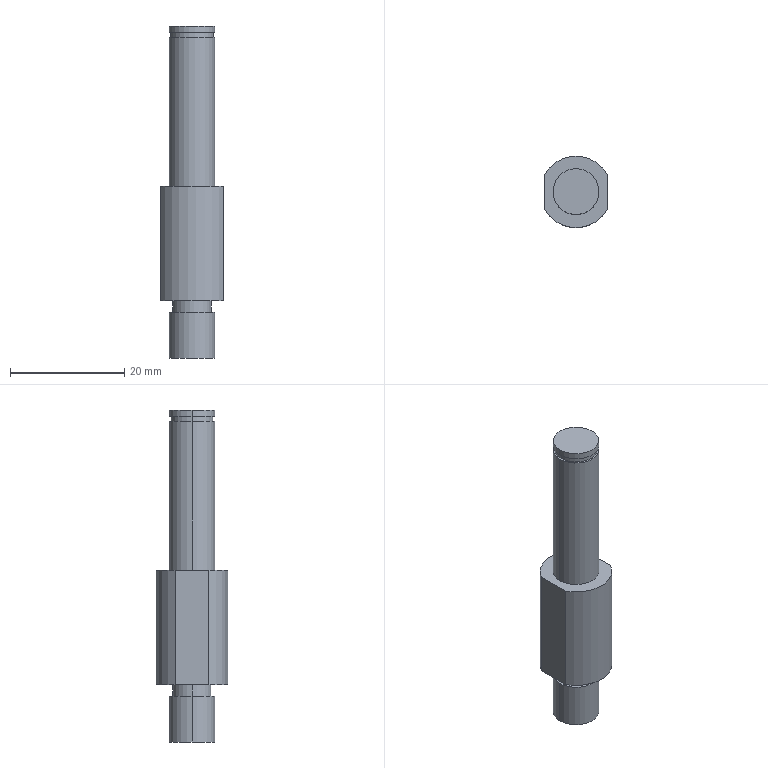Component | SolidWorks | JL001-03-03-1_JL001-03-03-001-1 | 1 solid | 21 faces | box 11 x 12.5 x 58 mm | volume 4210 mm3 | cylinder 12 | plane 9 | commonest cylinder face diameters 8 x6 6.8 x2 7.4 x2 12.5 x2
build123d program:
from build123d import *

# Parameters (mm, degrees)
SKETCH6_OUTSIDE_W   = 26.626
SKETCH6_OUTSIDE_H   = 26.626
SKETCH6_OUTSIDE_W_2 = 19.7
SKETCH6_OUTSIDE_H_2 = 11
CUT_EXTRUDE2_DEPTH  = 32.275


with BuildPart() as part:
    # Sketch1 → Revolve1 (revolve)
    with BuildSketch(Plane.XY, mode=Mode.PRIVATE) as revolve1_sk:
        Polygon((0, 58), (4, 58), (4, 56.9), (3.7, 56.9), (3.7, 56), (4, 56), (4, 30), (6.25, 30), (6.25, 10), (3.4, 10), (3.4, 8), (4, 8), (4, 0), (0, 0), align=None)
    revolve(revolve1_sk.sketch.rotate(Axis((0, 0, 0), (0, 1, 0)), 90), axis=Axis((0, 0, 0), (0, 1, 0)))

    # Sketch6 outside → Cut-Extrude2 (cut, through all)
    with BuildSketch(Plane(origin=(0, 30, 0), x_dir=(1, 0, 0), z_dir=(0, 1, 0))):
        Rectangle(SKETCH6_OUTSIDE_W, SKETCH6_OUTSIDE_H)
        Rectangle(SKETCH6_OUTSIDE_W_2, SKETCH6_OUTSIDE_H_2, mode=Mode.SUBTRACT)
    extrude(amount=-CUT_EXTRUDE2_DEPTH, mode=Mode.SUBTRACT)


solid = part.part

# Placed as in the assembly
solid = solid.moved(Location((15, 27.5, -2.5), (90, -90, 0)))
STEP:
#1=COLOUR_RGB('',0.7922,0.8196,0.9333);
#2=FILL_AREA_STYLE_COLOUR('',#1);
#3=FILL_AREA_STYLE('',(#2));
#4=SURFACE_STYLE_FILL_AREA(#3);
#5=SURFACE_SIDE_STYLE('',(#4));
#6=SURFACE_STYLE_USAGE(.BOTH.,#5);
#7=PRESENTATION_STYLE_ASSIGNMENT((#6));
#8=CARTESIAN_POINT('',(0.748,1.083,0.2165));
#9=VERTEX_POINT('',#8);
#10=CARTESIAN_POINT('',(0.4331,1.083,0.2165));
#11=VERTEX_POINT('',#10);
#12=CARTESIAN_POINT('',(0.5906,1.083,0.2165));
#13=DIRECTION('',(0.,0.,-1.));
#14=DIRECTION('',(1.,0.,0.));
#15=AXIS2_PLACEMENT_3D('',#12,#13,#14);
#16=CIRCLE('',#15,0.1575);
#17=EDGE_CURVE('',#9,#11,#16,.T.);
#18=ORIENTED_EDGE('',*,*,#17,.T.);
#19=CARTESIAN_POINT('',(0.4331,1.083,-0.09843));
#20=VERTEX_POINT('',#19);
#21=CARTESIAN_POINT('',(0.4331,1.083,-0.09843));
#22=DIRECTION('',(0.,0.,-1.));
#23=VECTOR('',#22,39.37);
#24=LINE('',#21,#23);
#25=EDGE_CURVE('',#11,#20,#24,.T.);
#26=ORIENTED_EDGE('',*,*,#25,.T.);
#27=CARTESIAN_POINT('',(0.748,1.083,-0.09843));
#28=VERTEX_POINT('',#27);
#29=CARTESIAN_POINT('',(0.5906,1.083,-0.09843));
#30=DIRECTION('',(0.,0.,-1.));
#31=DIRECTION('',(1.,0.,0.));
#32=AXIS2_PLACEMENT_3D('',#29,#30,#31);
#33=CIRCLE('',#32,0.1575);
#34=EDGE_CURVE('',#28,#20,#33,.T.);
#35=ORIENTED_EDGE('',*,*,#34,.F.);
#36=CARTESIAN_POINT('',(0.748,1.083,-0.09843));
#37=DIRECTION('',(0.,0.,-1.));
#38=VECTOR('',#37,39.37);
#39=LINE('',#36,#38);
#40=EDGE_CURVE('',#9,#28,#39,.T.);
#41=ORIENTED_EDGE('',*,*,#40,.F.);
#42=EDGE_LOOP('',(#18,#26,#35,#41));
#43=FACE_OUTER_BOUND('',#42,.T.);
#44=CARTESIAN_POINT('',(0.5906,1.083,-0.09843));
#45=DIRECTION('',(0.,0.,-1.));
#46=DIRECTION('',(1.,0.,0.));
#47=AXIS2_PLACEMENT_3D('',#44,#45,#46);
#48=CYLINDRICAL_SURFACE('',#47,0.1575);
#49=ADVANCED_FACE('',(#43),#48,.T.);
#50=CARTESIAN_POINT('',(0.7244,1.083,0.2953));
#51=VERTEX_POINT('',#50);
#52=CARTESIAN_POINT('',(0.4567,1.083,0.2953));
#53=VERTEX_POINT('',#52);
#54=CARTESIAN_POINT('',(0.5906,1.083,0.2953));
#55=DIRECTION('',(0.,0.,-1.));
#56=DIRECTION('',(1.,0.,0.));
#57=AXIS2_PLACEMENT_3D('',#54,#55,#56);
#58=CIRCLE('',#57,0.1339);
#59=EDGE_CURVE('',#51,#53,#58,.T.);
#60=ORIENTED_EDGE('',*,*,#59,.T.);
#61=CARTESIAN_POINT('',(0.4567,1.083,0.2165));
#62=VERTEX_POINT('',#61);
#63=CARTESIAN_POINT('',(0.4567,1.083,-0.09843));
#64=DIRECTION('',(0.,0.,-1.));
#65=VECTOR('',#64,39.37);
#66=LINE('',#63,#65);
#67=EDGE_CURVE('',#53,#62,#66,.T.);
#68=ORIENTED_EDGE('',*,*,#67,.T.);
#69=CARTESIAN_POINT('',(0.7244,1.083,0.2165));
#70=VERTEX_POINT('',#69);
#71=CARTESIAN_POINT('',(0.5906,1.083,0.2165));
#72=DIRECTION('',(0.,0.,-1.));
#73=DIRECTION('',(1.,0.,0.));
#74=AXIS2_PLACEMENT_3D('',#71,#72,#73);
#75=CIRCLE('',#74,0.1339);
#76=EDGE_CURVE('',#70,#62,#75,.T.);
#77=ORIENTED_EDGE('',*,*,#76,.F.);
#78=CARTESIAN_POINT('',(0.7244,1.083,-0.09843));
#79=DIRECTION('',(0.,0.,-1.));
#80=VECTOR('',#79,39.37);
#81=LINE('',#78,#80);
#82=EDGE_CURVE('',#51,#70,#81,.T.);
#83=ORIENTED_EDGE('',*,*,#82,.F.);
#84=EDGE_LOOP('',(#60,#68,#77,#83));
#85=FACE_OUTER_BOUND('',#84,.T.);
#86=CARTESIAN_POINT('',(0.5906,1.083,-0.09843));
#87=DIRECTION('',(0.,0.,-1.));
#88=DIRECTION('',(1.,0.,0.));
#89=AXIS2_PLACEMENT_3D('',#86,#87,#88);
#90=CYLINDRICAL_SURFACE('',#89,0.1339);
#91=ADVANCED_FACE('',(#85),#90,.T.);
#92=CARTESIAN_POINT('',(0.748,1.083,2.106));
#93=VERTEX_POINT('',#92);
#94=CARTESIAN_POINT('',(0.4331,1.083,2.106));
#95=VERTEX_POINT('',#94);
#96=CARTESIAN_POINT('',(0.5906,1.083,2.106));
#97=DIRECTION('',(0.,0.,-1.));
#98=DIRECTION('',(1.,0.,0.));
#99=AXIS2_PLACEMENT_3D('',#96,#97,#98);
#100=CIRCLE('',#99,0.1575);
#101=EDGE_CURVE('',#93,#95,#100,.T.);
#102=ORIENTED_EDGE('',*,*,#101,.T.);
#103=CARTESIAN_POINT('',(0.4331,1.083,1.083));
#104=VERTEX_POINT('',#103);
#105=CARTESIAN_POINT('',(0.4331,1.083,-0.09843));
#106=DIRECTION('',(0.,0.,-1.));
#107=VECTOR('',#106,39.37);
#108=LINE('',#105,#107);
#109=EDGE_CURVE('',#95,#104,#108,.T.);
#110=ORIENTED_EDGE('',*,*,#109,.T.);
#111=CARTESIAN_POINT('',(0.748,1.083,1.083));
#112=VERTEX_POINT('',#111);
#113=CARTESIAN_POINT('',(0.5906,1.083,1.083));
#114=DIRECTION('',(0.,0.,-1.));
#115=DIRECTION('',(1.,0.,0.));
#116=AXIS2_PLACEMENT_3D('',#113,#114,#115);
#117=CIRCLE('',#116,0.1575);
#118=EDGE_CURVE('',#112,#104,#117,.T.);
#119=ORIENTED_EDGE('',*,*,#118,.F.);
#120=CARTESIAN_POINT('',(0.748,1.083,-0.09843));
#121=DIRECTION('',(0.,0.,-1.));
#122=VECTOR('',#121,39.37);
#123=LINE('',#120,#122);
#124=EDGE_CURVE('',#93,#112,#123,.T.);
#125=ORIENTED_EDGE('',*,*,#124,.F.);
#126=EDGE_LOOP('',(#102,#110,#119,#125));
#127=FACE_OUTER_BOUND('',#126,.T.);
#128=CARTESIAN_POINT('',(0.5906,1.083,-0.09843));
#129=DIRECTION('',(0.,0.,-1.));
#130=DIRECTION('',(1.,0.,0.));
#131=AXIS2_PLACEMENT_3D('',#128,#129,#130);
#132=CYLINDRICAL_SURFACE('',#131,0.1575);
#133=ADVANCED_FACE('',(#127),#132,.T.);
#134=CARTESIAN_POINT('',(0.7362,1.083,2.142));
#135=VERTEX_POINT('',#134);
#136=CARTESIAN_POINT('',(0.4449,1.083,2.142));
#137=VERTEX_POINT('',#136);
#138=CARTESIAN_POINT('',(0.5906,1.083,2.142));
#139=DIRECTION('',(0.,0.,-1.));
#140=DIRECTION('',(1.,0.,0.));
#141=AXIS2_PLACEMENT_3D('',#138,#139,#140);
#142=CIRCLE('',#141,0.1457);
#143=EDGE_CURVE('',#135,#137,#142,.T.);
#144=ORIENTED_EDGE('',*,*,#143,.T.);
#145=CARTESIAN_POINT('',(0.4449,1.083,2.106));
#146=VERTEX_POINT('',#145);
#147=CARTESIAN_POINT('',(0.4449,1.083,-0.09843));
#148=DIRECTION('',(0.,0.,-1.));
#149=VECTOR('',#148,39.37);
#150=LINE('',#147,#149);
#151=EDGE_CURVE('',#137,#146,#150,.T.);
#152=ORIENTED_EDGE('',*,*,#151,.T.);
#153=CARTESIAN_POINT('',(0.7362,1.083,2.106));
#154=VERTEX_POINT('',#153);
#155=CARTESIAN_POINT('',(0.5906,1.083,2.106));
#156=DIRECTION('',(0.,0.,-1.));
#157=DIRECTION('',(1.,0.,0.));
#158=AXIS2_PLACEMENT_3D('',#155,#156,#157);
#159=CIRCLE('',#158,0.1457);
#160=EDGE_CURVE('',#154,#146,#159,.T.);
#161=ORIENTED_EDGE('',*,*,#160,.F.);
#162=CARTESIAN_POINT('',(0.7362,1.083,-0.09843));
#163=DIRECTION('',(0.,0.,-1.));
#164=VECTOR('',#163,39.37);
#165=LINE('',#162,#164);
#166=EDGE_CURVE('',#135,#154,#165,.T.);
#167=ORIENTED_EDGE('',*,*,#166,.F.);
#168=EDGE_LOOP('',(#144,#152,#161,#167));
#169=FACE_OUTER_BOUND('',#168,.T.);
#170=CARTESIAN_POINT('',(0.5906,1.083,-0.09843));
#171=DIRECTION('',(0.,0.,-1.));
#172=DIRECTION('',(1.,0.,0.));
#173=AXIS2_PLACEMENT_3D('',#170,#171,#172);
#174=CYLINDRICAL_SURFACE('',#173,0.1457);
#175=ADVANCED_FACE('',(#169),#174,.T.);
#176=CARTESIAN_POINT('',(0.748,1.083,2.185));
#177=VERTEX_POINT('',#176);
#178=CARTESIAN_POINT('',(0.4331,1.083,2.185));
#179=VERTEX_POINT('',#178);
#180=CARTESIAN_POINT('',(0.5906,1.083,2.185));
#181=DIRECTION('',(0.,0.,-1.));
#182=DIRECTION('',(1.,0.,0.));
#183=AXIS2_PLACEMENT_3D('',#180,#181,#182);
#184=CIRCLE('',#183,0.1575);
#185=EDGE_CURVE('',#177,#179,#184,.T.);
#186=ORIENTED_EDGE('',*,*,#185,.T.);
#187=CARTESIAN_POINT('',(0.4331,1.083,2.142));
#188=VERTEX_POINT('',#187);
#189=CARTESIAN_POINT('',(0.4331,1.083,-0.09843));
#190=DIRECTION('',(0.,0.,-1.));
#191=VECTOR('',#190,39.37);
#192=LINE('',#189,#191);
#193=EDGE_CURVE('',#179,#188,#192,.T.);
#194=ORIENTED_EDGE('',*,*,#193,.T.);
#195=CARTESIAN_POINT('',(0.748,1.083,2.142));
#196=VERTEX_POINT('',#195);
#197=CARTESIAN_POINT('',(0.5906,1.083,2.142));
#198=DIRECTION('',(0.,0.,-1.));
#199=DIRECTION('',(1.,0.,0.));
#200=AXIS2_PLACEMENT_3D('',#197,#198,#199);
#201=CIRCLE('',#200,0.1575);
#202=EDGE_CURVE('',#196,#188,#201,.T.);
#203=ORIENTED_EDGE('',*,*,#202,.F.);
#204=CARTESIAN_POINT('',(0.748,1.083,-0.09843));
#205=DIRECTION('',(0.,0.,-1.));
#206=VECTOR('',#205,39.37);
#207=LINE('',#204,#206);
#208=EDGE_CURVE('',#177,#196,#207,.T.);
#209=ORIENTED_EDGE('',*,*,#208,.F.);
#210=EDGE_LOOP('',(#186,#194,#203,#209));
#211=FACE_OUTER_BOUND('',#210,.T.);
#212=CARTESIAN_POINT('',(0.5906,1.083,-0.09843));
#213=DIRECTION('',(0.,0.,-1.));
#214=DIRECTION('',(1.,0.,0.));
#215=AXIS2_PLACEMENT_3D('',#212,#213,#214);
#216=CYLINDRICAL_SURFACE('',#215,0.1575);
#217=ADVANCED_FACE('',(#211),#216,.T.);
#218=ORIENTED_EDGE('',*,*,#118,.T.);
#219=CARTESIAN_POINT('',(0.5906,1.083,1.083));
#220=DIRECTION('',(0.,0.,-1.));
#221=DIRECTION('',(1.,0.,0.));
#222=AXIS2_PLACEMENT_3D('',#219,#220,#221);
#223=CIRCLE('',#222,0.1575);
#224=EDGE_CURVE('',#104,#112,#223,.T.);
#225=ORIENTED_EDGE('',*,*,#224,.T.);
#226=EDGE_LOOP('',(#218,#225));
#227=FACE_BOUND('',#226,.T.);
#228=CARTESIAN_POINT('',(0.374,1.2,1.083));
#229=VERTEX_POINT('',#228);
#230=CARTESIAN_POINT('',(0.8071,1.2,1.083));
#231=VERTEX_POINT('',#230);
#232=CARTESIAN_POINT('',(0.5906,1.083,1.083));
#233=DIRECTION('',(0.,0.,-1.));
#234=DIRECTION('',(1.,0.,0.));
#235=AXIS2_PLACEMENT_3D('',#232,#233,#234);
#236=CIRCLE('',#235,0.2461);
#237=EDGE_CURVE('',#229,#231,#236,.T.);
#238=ORIENTED_EDGE('',*,*,#237,.F.);
#239=CARTESIAN_POINT('',(0.374,0.9658,1.083));
#240=VERTEX_POINT('',#239);
#241=CARTESIAN_POINT('',(0.374,1.47,1.083));
#242=DIRECTION('',(0.,-1.,0.));
#243=VECTOR('',#242,39.37);
#244=LINE('',#241,#243);
#245=EDGE_CURVE('',#229,#240,#244,.T.);
#246=ORIENTED_EDGE('',*,*,#245,.T.);
#247=CARTESIAN_POINT('',(0.8071,0.9658,1.083));
#248=VERTEX_POINT('',#247);
#249=CARTESIAN_POINT('',(0.5906,1.083,1.083));
#250=DIRECTION('',(0.,0.,-1.));
#251=DIRECTION('',(1.,0.,0.));
#252=AXIS2_PLACEMENT_3D('',#249,#250,#251);
#253=CIRCLE('',#252,0.2461);
#254=EDGE_CURVE('',#248,#240,#253,.T.);
#255=ORIENTED_EDGE('',*,*,#254,.F.);
#256=CARTESIAN_POINT('',(0.8071,1.47,1.083));
#257=DIRECTION('',(-0.,1.,0.));
#258=VECTOR('',#257,39.37);
#259=LINE('',#256,#258);
#260=EDGE_CURVE('',#248,#231,#259,.T.);
#261=ORIENTED_EDGE('',*,*,#260,.T.);
#262=EDGE_LOOP('',(#238,#246,#255,#261));
#263=FACE_OUTER_BOUND('',#262,.T.);
#264=CARTESIAN_POINT('',(0.5906,0.9252,1.083));
#265=DIRECTION('',(0.,0.,1.));
#266=DIRECTION('',(-1.,-0.,0.));
#267=AXIS2_PLACEMENT_3D('',#264,#265,#266);
#268=PLANE('',#267);
#269=ADVANCED_FACE('',(#227,#263),#268,.T.);
#270=CARTESIAN_POINT('',(0.374,1.2,0.2953));
#271=VERTEX_POINT('',#270);
#272=CARTESIAN_POINT('',(0.8071,1.2,0.2953));
#273=VERTEX_POINT('',#272);
#274=CARTESIAN_POINT('',(0.5906,1.083,0.2953));
#275=DIRECTION('',(0.,0.,-1.));
#276=DIRECTION('',(1.,0.,0.));
#277=AXIS2_PLACEMENT_3D('',#274,#275,#276);
#278=CIRCLE('',#277,0.2461);
#279=EDGE_CURVE('',#271,#273,#278,.T.);
#280=ORIENTED_EDGE('',*,*,#279,.F.);
#281=CARTESIAN_POINT('',(0.374,1.2,-0.09843));
#282=DIRECTION('',(0.,0.,1.));
#283=VECTOR('',#282,39.37);
#284=LINE('',#281,#283);
#285=EDGE_CURVE('',#271,#229,#284,.T.);
#286=ORIENTED_EDGE('',*,*,#285,.T.);
#287=ORIENTED_EDGE('',*,*,#237,.T.);
#288=CARTESIAN_POINT('',(0.8071,1.2,-0.09843));
#289=DIRECTION('',(0.,0.,-1.));
#290=VECTOR('',#289,39.37);
#291=LINE('',#288,#290);
#292=EDGE_CURVE('',#231,#273,#291,.T.);
#293=ORIENTED_EDGE('',*,*,#292,.T.);
#294=EDGE_LOOP('',(#280,#286,#287,#293));
#295=FACE_OUTER_BOUND('',#294,.T.);
#296=CARTESIAN_POINT('',(0.5906,1.083,-0.09843));
#297=DIRECTION('',(0.,0.,-1.));
#298=DIRECTION('',(1.,0.,0.));
#299=AXIS2_PLACEMENT_3D('',#296,#297,#298);
#300=CYLINDRICAL_SURFACE('',#299,0.2461);
#301=ADVANCED_FACE('',(#295),#300,.T.);
#302=ORIENTED_EDGE('',*,*,#254,.T.);
#303=CARTESIAN_POINT('',(0.374,0.9658,0.2953));
#304=VERTEX_POINT('',#303);
#305=CARTESIAN_POINT('',(0.374,0.9658,-0.09843));
#306=DIRECTION('',(0.,0.,-1.));
#307=VECTOR('',#306,39.37);
#308=LINE('',#305,#307);
#309=EDGE_CURVE('',#240,#304,#308,.T.);
#310=ORIENTED_EDGE('',*,*,#309,.T.);
#311=CARTESIAN_POINT('',(0.8071,0.9658,0.2953));
#312=VERTEX_POINT('',#311);
#313=CARTESIAN_POINT('',(0.5906,1.083,0.2953));
#314=DIRECTION('',(0.,0.,-1.));
#315=DIRECTION('',(1.,0.,0.));
#316=AXIS2_PLACEMENT_3D('',#313,#314,#315);
#317=CIRCLE('',#316,0.2461);
#318=EDGE_CURVE('',#312,#304,#317,.T.);
#319=ORIENTED_EDGE('',*,*,#318,.F.);
#320=CARTESIAN_POINT('',(0.8071,0.9658,-0.09843));
#321=DIRECTION('',(0.,0.,1.));
#322=VECTOR('',#321,39.37);
#323=LINE('',#320,#322);
#324=EDGE_CURVE('',#312,#248,#323,.T.);
#325=ORIENTED_EDGE('',*,*,#324,.T.);
#326=EDGE_LOOP('',(#302,#310,#319,#325));
#327=FACE_OUTER_BOUND('',#326,.T.);
#328=CARTESIAN_POINT('',(0.5906,1.083,-0.09843));
#329=DIRECTION('',(0.,0.,-1.));
#330=DIRECTION('',(1.,0.,0.));
#331=AXIS2_PLACEMENT_3D('',#328,#329,#330);
#332=CYLINDRICAL_SURFACE('',#331,0.2461);
#333=ADVANCED_FACE('',(#327),#332,.T.);
#334=ORIENTED_EDGE('',*,*,#59,.F.);
#335=CARTESIAN_POINT('',(0.5906,1.083,0.2953));
#336=DIRECTION('',(0.,0.,-1.));
#337=DIRECTION('',(1.,0.,0.));
#338=AXIS2_PLACEMENT_3D('',#335,#336,#337);
#339=CIRCLE('',#338,0.1339);
#340=EDGE_CURVE('',#53,#51,#339,.T.);
#341=ORIENTED_EDGE('',*,*,#340,.F.);
#342=EDGE_LOOP('',(#334,#341));
#343=FACE_BOUND('',#342,.T.);
#344=ORIENTED_EDGE('',*,*,#318,.T.);
#345=CARTESIAN_POINT('',(0.374,0.8366,0.2953));
#346=DIRECTION('',(-0.,1.,0.));
#347=VECTOR('',#346,39.37);
#348=LINE('',#345,#347);
#349=EDGE_CURVE('',#304,#271,#348,.T.);
#350=ORIENTED_EDGE('',*,*,#349,.T.);
#351=ORIENTED_EDGE('',*,*,#279,.T.);
#352=CARTESIAN_POINT('',(0.8071,0.8366,0.2953));
#353=DIRECTION('',(0.,-1.,0.));
#354=VECTOR('',#353,39.37);
#355=LINE('',#352,#354);
#356=EDGE_CURVE('',#273,#312,#355,.T.);
#357=ORIENTED_EDGE('',*,*,#356,.T.);
#358=EDGE_LOOP('',(#344,#350,#351,#357));
#359=FACE_OUTER_BOUND('',#358,.T.);
#360=CARTESIAN_POINT('',(0.5906,0.8366,0.2953));
#361=DIRECTION('',(0.,0.,-1.));
#362=DIRECTION('',(1.,0.,0.));
#363=AXIS2_PLACEMENT_3D('',#360,#361,#362);
#364=PLANE('',#363);
#365=ADVANCED_FACE('',(#343,#359),#364,.T.);
#366=ORIENTED_EDGE('',*,*,#185,.F.);
#367=CARTESIAN_POINT('',(0.5906,1.083,2.185));
#368=DIRECTION('',(0.,0.,-1.));
#369=DIRECTION('',(1.,0.,0.));
#370=AXIS2_PLACEMENT_3D('',#367,#368,#369);
#371=CIRCLE('',#370,0.1575);
#372=EDGE_CURVE('',#179,#177,#371,.T.);
#373=ORIENTED_EDGE('',*,*,#372,.F.);
#374=EDGE_LOOP('',(#366,#373));
#375=FACE_OUTER_BOUND('',#374,.T.);
#376=CARTESIAN_POINT('',(0.5906,1.083,2.185));
#377=DIRECTION('',(0.,0.,1.));
#378=DIRECTION('',(-1.,-0.,0.));
#379=AXIS2_PLACEMENT_3D('',#376,#377,#378);
#380=PLANE('',#379);
#381=ADVANCED_FACE('',(#375),#380,.T.);
#382=ORIENTED_EDGE('',*,*,#193,.F.);
#383=ORIENTED_EDGE('',*,*,#372,.T.);
#384=ORIENTED_EDGE('',*,*,#208,.T.);
#385=CARTESIAN_POINT('',(0.5906,1.083,2.142));
#386=DIRECTION('',(0.,0.,-1.));
#387=DIRECTION('',(1.,0.,0.));
#388=AXIS2_PLACEMENT_3D('',#385,#386,#387);
#389=CIRCLE('',#388,0.1575);
#390=EDGE_CURVE('',#188,#196,#389,.T.);
#391=ORIENTED_EDGE('',*,*,#390,.F.);
#392=EDGE_LOOP('',(#382,#383,#384,#391));
#393=FACE_OUTER_BOUND('',#392,.T.);
#394=CARTESIAN_POINT('',(0.5906,1.083,-0.09843));
#395=DIRECTION('',(0.,0.,-1.));
#396=DIRECTION('',(1.,0.,0.));
#397=AXIS2_PLACEMENT_3D('',#394,#395,#396);
#398=CYLINDRICAL_SURFACE('',#397,0.1575);
#399=ADVANCED_FACE('',(#393),#398,.T.);
#400=ORIENTED_EDGE('',*,*,#202,.T.);
#401=ORIENTED_EDGE('',*,*,#390,.T.);
#402=EDGE_LOOP('',(#400,#401));
#403=FACE_OUTER_BOUND('',#402,.T.);
#404=ORIENTED_EDGE('',*,*,#143,.F.);
#405=CARTESIAN_POINT('',(0.5906,1.083,2.142));
#406=DIRECTION('',(0.,0.,-1.));
#407=DIRECTION('',(1.,0.,0.));
#408=AXIS2_PLACEMENT_3D('',#405,#406,#407);
#409=CIRCLE('',#408,0.1457);
#410=EDGE_CURVE('',#137,#135,#409,.T.);
#411=ORIENTED_EDGE('',*,*,#410,.F.);
#412=EDGE_LOOP('',(#404,#411));
#413=FACE_BOUND('',#412,.T.);
#414=CARTESIAN_POINT('',(0.5906,0.9252,2.142));
#415=DIRECTION('',(0.,0.,-1.));
#416=DIRECTION('',(1.,0.,0.));
#417=AXIS2_PLACEMENT_3D('',#414,#415,#416);
#418=PLANE('',#417);
#419=ADVANCED_FACE('',(#403,#413),#418,.T.);
#420=ORIENTED_EDGE('',*,*,#151,.F.);
#421=ORIENTED_EDGE('',*,*,#410,.T.);
#422=ORIENTED_EDGE('',*,*,#166,.T.);
#423=CARTESIAN_POINT('',(0.5906,1.083,2.106));
#424=DIRECTION('',(0.,0.,-1.));
#425=DIRECTION('',(1.,0.,0.));
#426=AXIS2_PLACEMENT_3D('',#423,#424,#425);
#427=CIRCLE('',#426,0.1457);
#428=EDGE_CURVE('',#146,#154,#427,.T.);
#429=ORIENTED_EDGE('',*,*,#428,.F.);
#430=EDGE_LOOP('',(#420,#421,#422,#429));
#431=FACE_OUTER_BOUND('',#430,.T.);
#432=CARTESIAN_POINT('',(0.5906,1.083,-0.09843));
#433=DIRECTION('',(0.,0.,-1.));
#434=DIRECTION('',(1.,0.,0.));
#435=AXIS2_PLACEMENT_3D('',#432,#433,#434);
#436=CYLINDRICAL_SURFACE('',#435,0.1457);
#437=ADVANCED_FACE('',(#431),#436,.T.);
#438=ORIENTED_EDGE('',*,*,#160,.T.);
#439=ORIENTED_EDGE('',*,*,#428,.T.);
#440=EDGE_LOOP('',(#438,#439));
#441=FACE_BOUND('',#440,.T.);
#442=ORIENTED_EDGE('',*,*,#101,.F.);
#443=CARTESIAN_POINT('',(0.5906,1.083,2.106));
#444=DIRECTION('',(0.,0.,-1.));
#445=DIRECTION('',(1.,0.,0.));
#446=AXIS2_PLACEMENT_3D('',#443,#444,#445);
#447=CIRCLE('',#446,0.1575);
#448=EDGE_CURVE('',#95,#93,#447,.T.);
#449=ORIENTED_EDGE('',*,*,#448,.F.);
#450=EDGE_LOOP('',(#442,#449));
#451=FACE_OUTER_BOUND('',#450,.T.);
#452=CARTESIAN_POINT('',(0.5906,0.937,2.106));
#453=DIRECTION('',(0.,0.,1.));
#454=DIRECTION('',(-1.,-0.,0.));
#455=AXIS2_PLACEMENT_3D('',#452,#453,#454);
#456=PLANE('',#455);
#457=ADVANCED_FACE('',(#441,#451),#456,.T.);
#458=ORIENTED_EDGE('',*,*,#109,.F.);
#459=ORIENTED_EDGE('',*,*,#448,.T.);
#460=ORIENTED_EDGE('',*,*,#124,.T.);
#461=ORIENTED_EDGE('',*,*,#224,.F.);
#462=EDGE_LOOP('',(#458,#459,#460,#461));
#463=FACE_OUTER_BOUND('',#462,.T.);
#464=CARTESIAN_POINT('',(0.5906,1.083,-0.09843));
#465=DIRECTION('',(0.,0.,-1.));
#466=DIRECTION('',(1.,0.,0.));
#467=AXIS2_PLACEMENT_3D('',#464,#465,#466);
#468=CYLINDRICAL_SURFACE('',#467,0.1575);
#469=ADVANCED_FACE('',(#463),#468,.T.);
#470=ORIENTED_EDGE('',*,*,#67,.F.);
#471=ORIENTED_EDGE('',*,*,#340,.T.);
#472=ORIENTED_EDGE('',*,*,#82,.T.);
#473=CARTESIAN_POINT('',(0.5906,1.083,0.2165));
#474=DIRECTION('',(0.,0.,-1.));
#475=DIRECTION('',(1.,0.,0.));
#476=AXIS2_PLACEMENT_3D('',#473,#474,#475);
#477=CIRCLE('',#476,0.1339);
#478=EDGE_CURVE('',#62,#70,#477,.T.);
#479=ORIENTED_EDGE('',*,*,#478,.F.);
#480=EDGE_LOOP('',(#470,#471,#472,#479));
#481=FACE_OUTER_BOUND('',#480,.T.);
#482=CARTESIAN_POINT('',(0.5906,1.083,-0.09843));
#483=DIRECTION('',(0.,0.,-1.));
#484=DIRECTION('',(1.,0.,0.));
#485=AXIS2_PLACEMENT_3D('',#482,#483,#484);
#486=CYLINDRICAL_SURFACE('',#485,0.1339);
#487=ADVANCED_FACE('',(#481),#486,.T.);
#488=ORIENTED_EDGE('',*,*,#76,.T.);
#489=ORIENTED_EDGE('',*,*,#478,.T.);
#490=EDGE_LOOP('',(#488,#489));
#491=FACE_BOUND('',#490,.T.);
#492=ORIENTED_EDGE('',*,*,#17,.F.);
#493=CARTESIAN_POINT('',(0.5906,1.083,0.2165));
#494=DIRECTION('',(0.,0.,-1.));
#495=DIRECTION('',(1.,0.,0.));
#496=AXIS2_PLACEMENT_3D('',#493,#494,#495);
#497=CIRCLE('',#496,0.1575);
#498=EDGE_CURVE('',#11,#9,#497,.T.);
#499=ORIENTED_EDGE('',*,*,#498,.F.);
#500=EDGE_LOOP('',(#492,#499));
#501=FACE_OUTER_BOUND('',#500,.T.);
#502=CARTESIAN_POINT('',(0.5906,0.9488,0.2165));
#503=DIRECTION('',(0.,0.,1.));
#504=DIRECTION('',(-1.,-0.,0.));
#505=AXIS2_PLACEMENT_3D('',#502,#503,#504);
#506=PLANE('',#505);
#507=ADVANCED_FACE('',(#491,#501),#506,.T.);
#508=ORIENTED_EDGE('',*,*,#25,.F.);
#509=ORIENTED_EDGE('',*,*,#498,.T.);
#510=ORIENTED_EDGE('',*,*,#40,.T.);
#511=CARTESIAN_POINT('',(0.5906,1.083,-0.09843));
#512=DIRECTION('',(0.,0.,-1.));
#513=DIRECTION('',(1.,0.,0.));
#514=AXIS2_PLACEMENT_3D('',#511,#512,#513);
#515=CIRCLE('',#514,0.1575);
#516=EDGE_CURVE('',#20,#28,#515,.T.);
#517=ORIENTED_EDGE('',*,*,#516,.F.);
#518=EDGE_LOOP('',(#508,#509,#510,#517));
#519=FACE_OUTER_BOUND('',#518,.T.);
#520=CARTESIAN_POINT('',(0.5906,1.083,-0.09843));
#521=DIRECTION('',(0.,0.,-1.));
#522=DIRECTION('',(1.,0.,0.));
#523=AXIS2_PLACEMENT_3D('',#520,#521,#522);
#524=CYLINDRICAL_SURFACE('',#523,0.1575);
#525=ADVANCED_FACE('',(#519),#524,.T.);
#526=ORIENTED_EDGE('',*,*,#34,.T.);
#527=ORIENTED_EDGE('',*,*,#516,.T.);
#528=EDGE_LOOP('',(#526,#527));
#529=FACE_OUTER_BOUND('',#528,.T.);
#530=CARTESIAN_POINT('',(0.5906,0.9252,-0.09843));
#531=DIRECTION('',(0.,0.,-1.));
#532=DIRECTION('',(1.,0.,0.));
#533=AXIS2_PLACEMENT_3D('',#530,#531,#532);
#534=PLANE('',#533);
#535=ADVANCED_FACE('',(#529),#534,.T.);
#536=ORIENTED_EDGE('',*,*,#356,.F.);
#537=ORIENTED_EDGE('',*,*,#292,.F.);
#538=ORIENTED_EDGE('',*,*,#260,.F.);
#539=ORIENTED_EDGE('',*,*,#324,.F.);
#540=EDGE_LOOP('',(#536,#537,#538,#539));
#541=FACE_OUTER_BOUND('',#540,.T.);
#542=CARTESIAN_POINT('',(0.8071,1.47,-0.09843));
#543=DIRECTION('',(1.,0.,0.));
#544=DIRECTION('',(-0.,1.,0.));
#545=AXIS2_PLACEMENT_3D('',#542,#543,#544);
#546=PLANE('',#545);
#547=ADVANCED_FACE('',(#541),#546,.T.);
#548=ORIENTED_EDGE('',*,*,#349,.F.);
#549=ORIENTED_EDGE('',*,*,#309,.F.);
#550=ORIENTED_EDGE('',*,*,#245,.F.);
#551=ORIENTED_EDGE('',*,*,#285,.F.);
#552=EDGE_LOOP('',(#548,#549,#550,#551));
#553=FACE_OUTER_BOUND('',#552,.T.);
#554=CARTESIAN_POINT('',(0.374,1.47,-0.09843));
#555=DIRECTION('',(-1.,-0.,0.));
#556=DIRECTION('',(0.,-1.,0.));
#557=AXIS2_PLACEMENT_3D('',#554,#555,#556);
#558=PLANE('',#557);
#559=ADVANCED_FACE('',(#553),#558,.T.);
#560=CLOSED_SHELL('',(#49,#91,#133,#175,#217,#269,#301,#333,#365,#381,#399,#419,#437,#457,#469,#487,#507,#525,#535,#547,#559));
#561=MANIFOLD_SOLID_BREP('',#560);
#562=STYLED_ITEM('',(#7),#561);
#563=PRESENTATION_LAYER_ASSIGNMENT('','',(#562));
#564=(LENGTH_UNIT()NAMED_UNIT(*)SI_UNIT($,.METRE.));
#565=LENGTH_MEASURE_WITH_UNIT(LENGTH_MEASURE(0.0254),#564);
#566=DIMENSIONAL_EXPONENTS(1.,0.,0.,0.,0.,0.,0.);
#567=(CONVERSION_BASED_UNIT('',#565)LENGTH_UNIT()NAMED_UNIT(#566));
#568=UNCERTAINTY_MEASURE_WITH_UNIT(LENGTH_MEASURE(0.00001),#567,'','');
#569=(NAMED_UNIT(*)PLANE_ANGLE_UNIT()SI_UNIT($,.RADIAN.));
#570=(NAMED_UNIT(*)SI_UNIT($,.STERADIAN.)SOLID_ANGLE_UNIT());
#571=(GEOMETRIC_REPRESENTATION_CONTEXT(3)GLOBAL_UNCERTAINTY_ASSIGNED_CONTEXT((#568))GLOBAL_UNIT_ASSIGNED_CONTEXT((#567,#569,#570))REPRESENTATION_CONTEXT('',''));
#572=MECHANICAL_DESIGN_GEOMETRIC_PRESENTATION_REPRESENTATION('',(#562),#571);
#573=CARTESIAN_POINT('',(0.,0.,0.));
#574=DIRECTION('',(0.,0.,1.));
#575=DIRECTION('',(1.,0.,0.));
#576=AXIS2_PLACEMENT_3D('',#573,#574,#575);
#577=(LENGTH_UNIT()NAMED_UNIT(*)SI_UNIT($,.METRE.));
#578=LENGTH_MEASURE_WITH_UNIT(LENGTH_MEASURE(0.0254),#577);
#579=DIMENSIONAL_EXPONENTS(1.,0.,0.,0.,0.,0.,0.);
#580=(CONVERSION_BASED_UNIT('',#578)LENGTH_UNIT()NAMED_UNIT(#579));
#581=UNCERTAINTY_MEASURE_WITH_UNIT(LENGTH_MEASURE(0.00001),#580,'','');
#582=(NAMED_UNIT(*)PLANE_ANGLE_UNIT()SI_UNIT($,.RADIAN.));
#583=(NAMED_UNIT(*)SI_UNIT($,.STERADIAN.)SOLID_ANGLE_UNIT());
#584=(GEOMETRIC_REPRESENTATION_CONTEXT(3)GLOBAL_UNCERTAINTY_ASSIGNED_CONTEXT((#581))GLOBAL_UNIT_ASSIGNED_CONTEXT((#580,#582,#583))REPRESENTATION_CONTEXT('',''));
#585=ADVANCED_BREP_SHAPE_REPRESENTATION('',(#561,#576),#584);